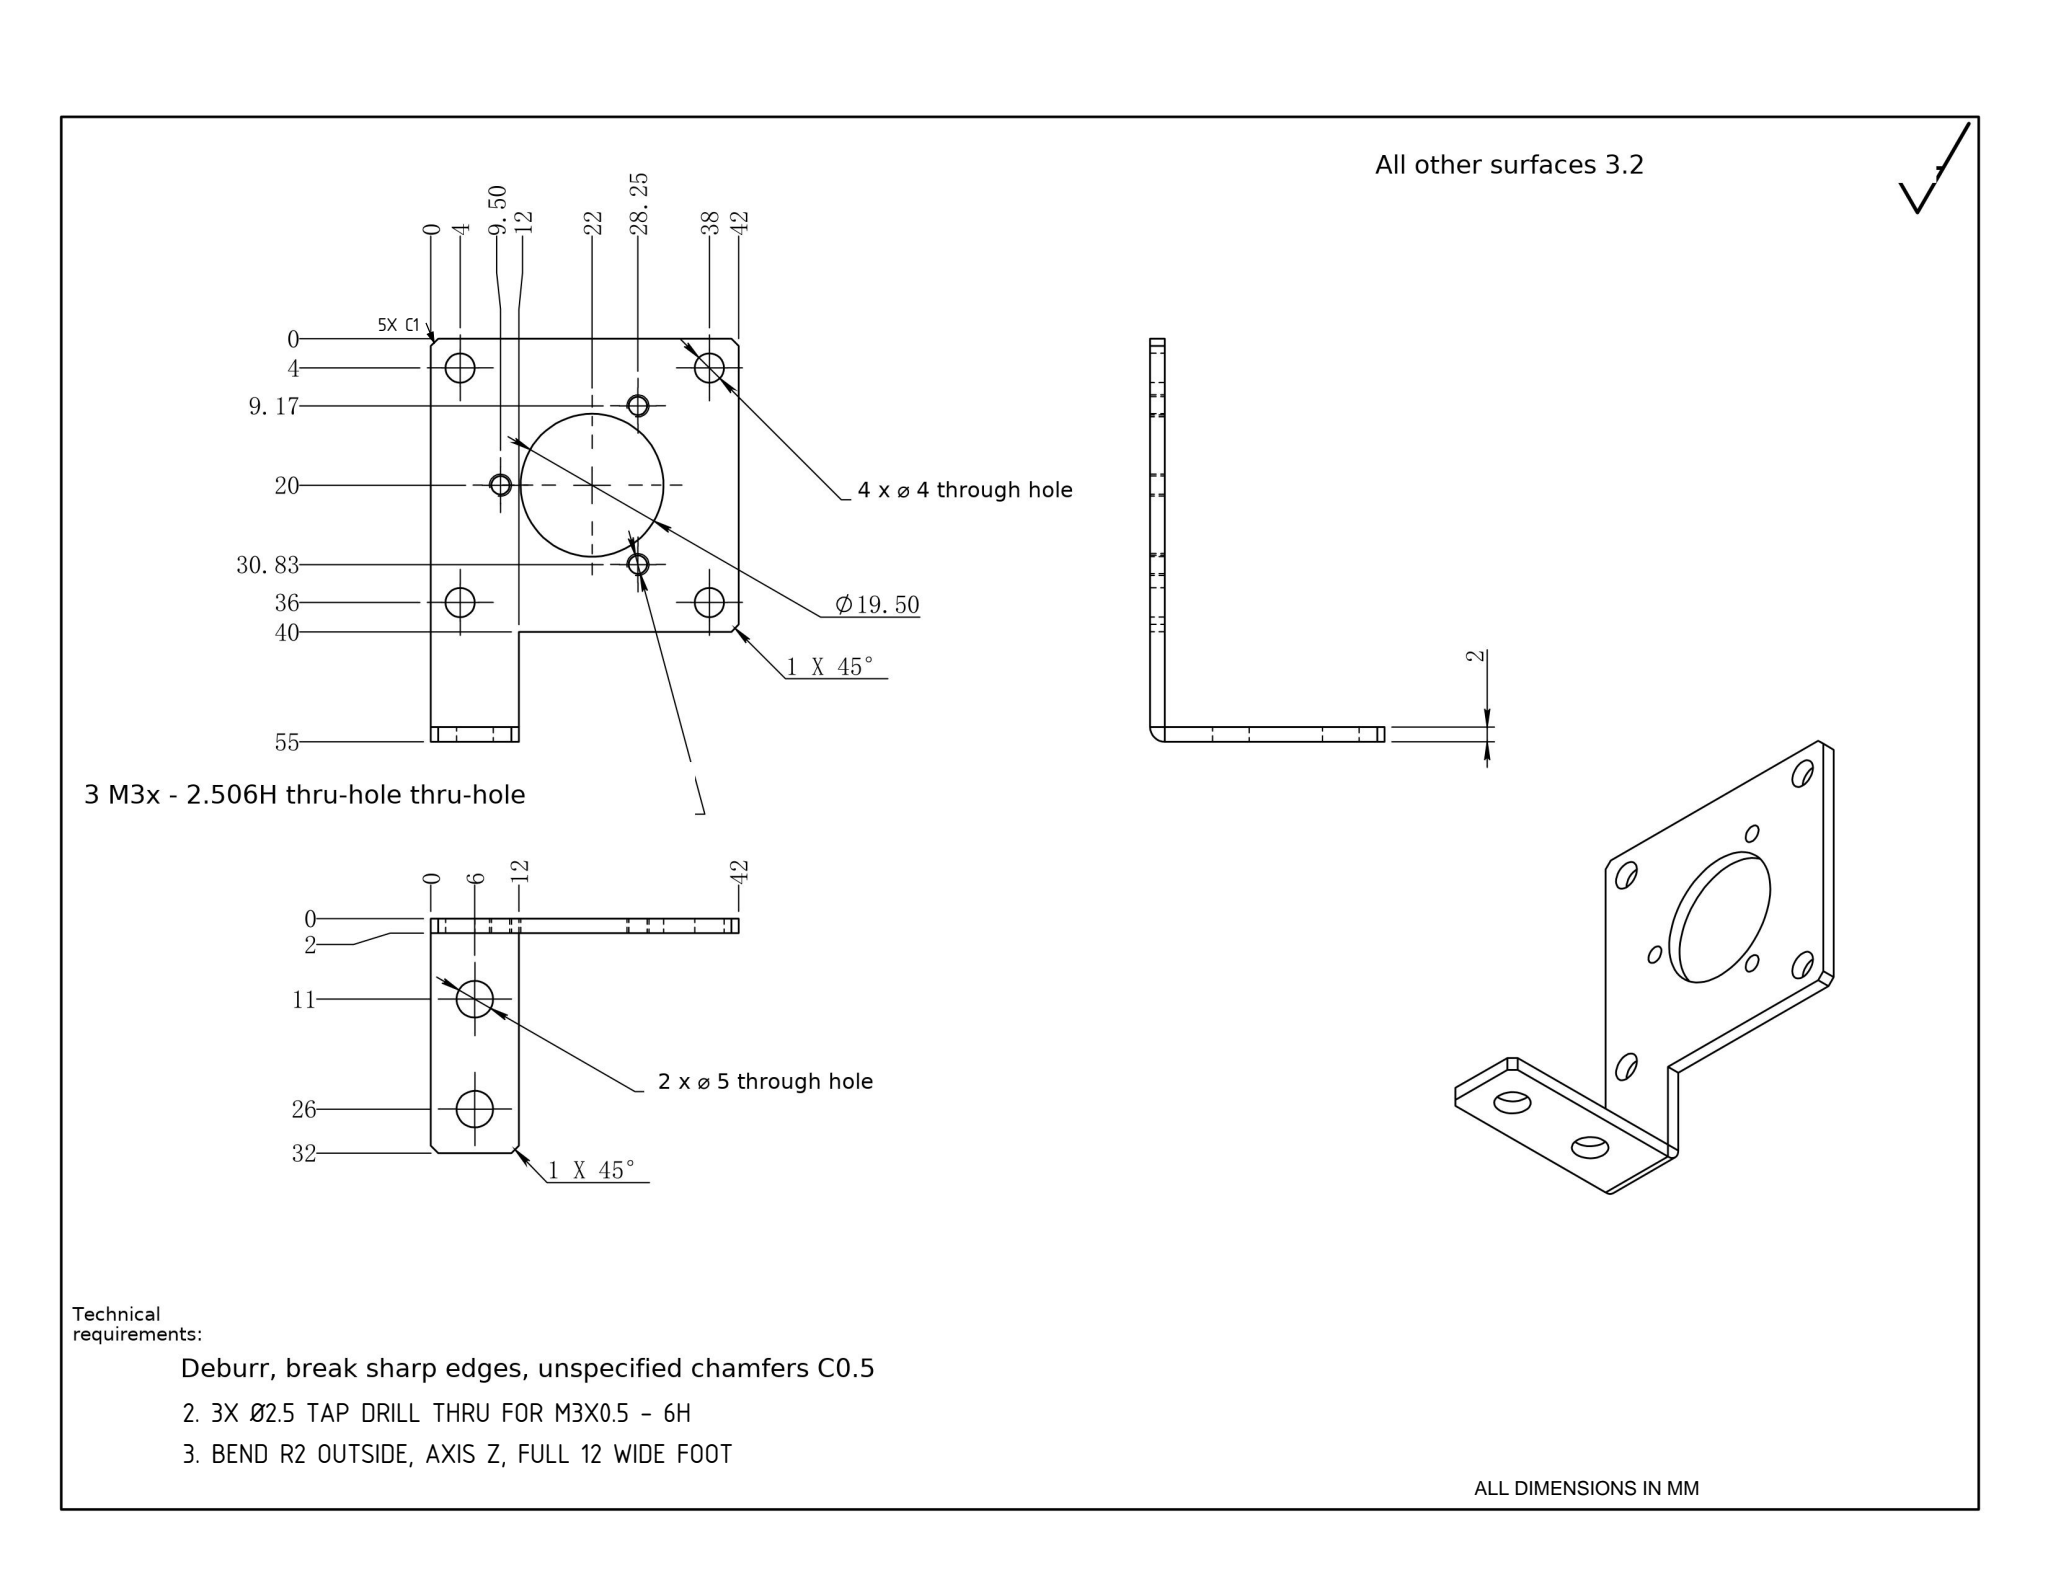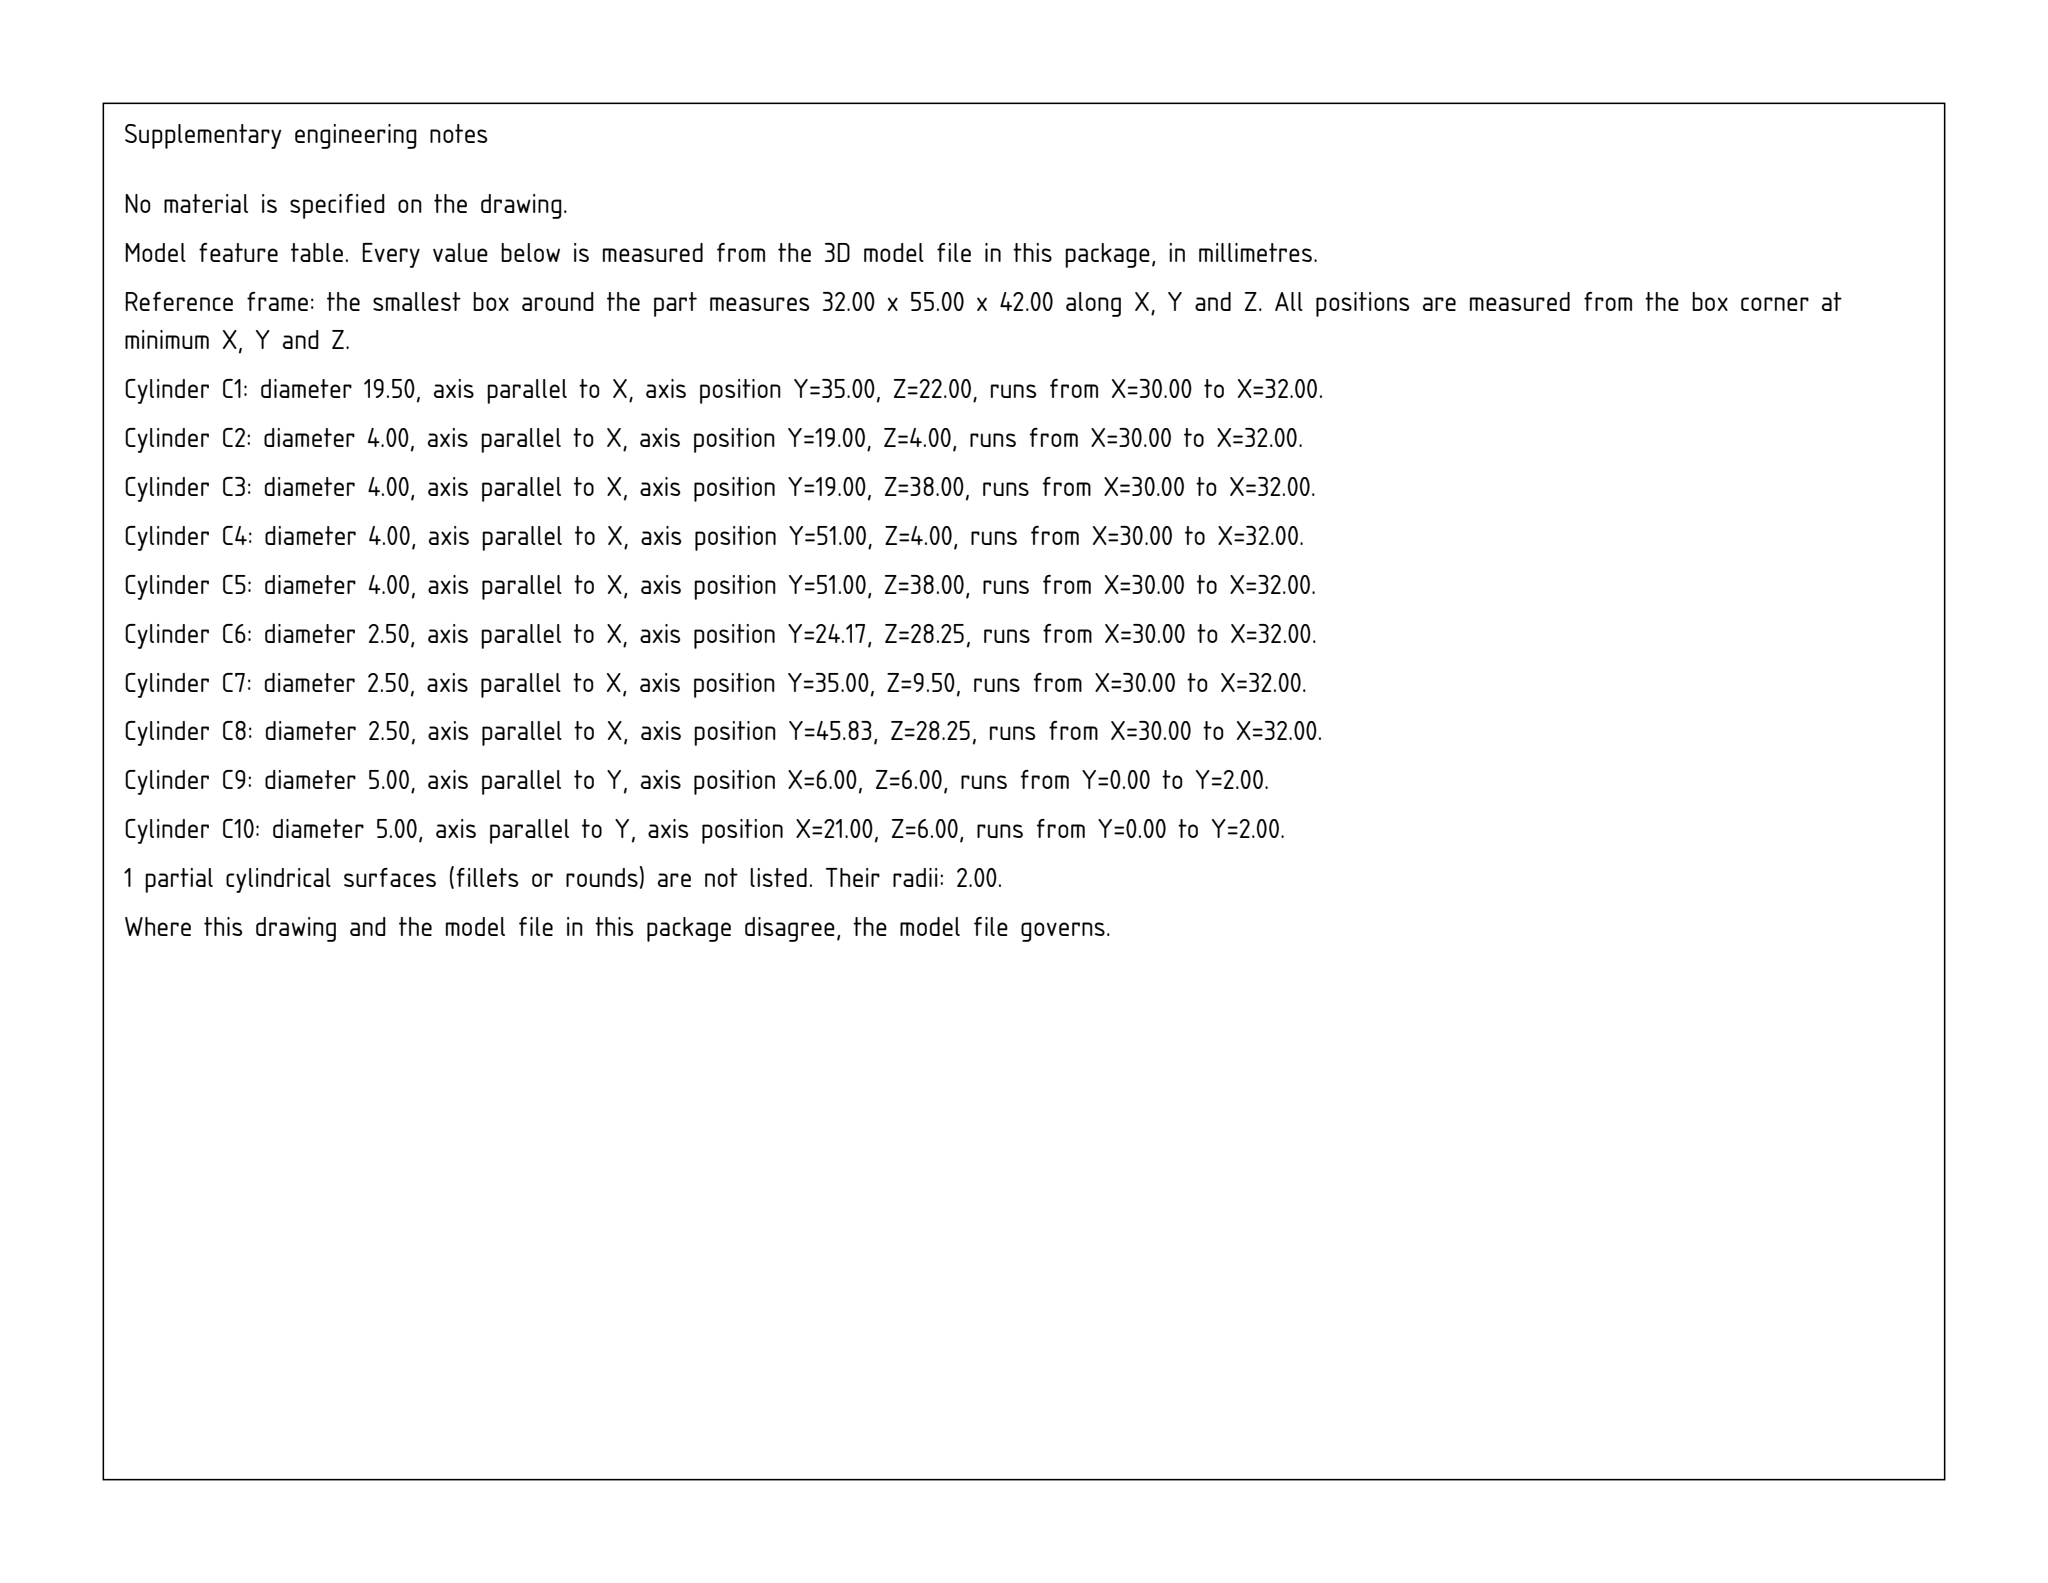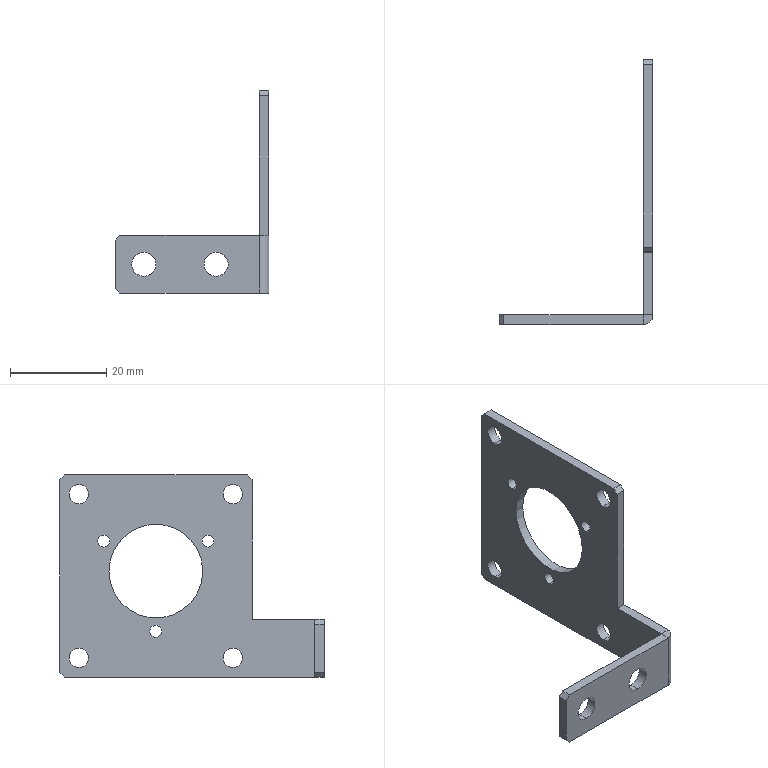Part | SolidWorks | mm | 1 solid | 40 faces | box 32 x 55 x 42 mm | volume 3619 mm3 | cylinder 21 | plane 19 | commonest cylinder face diameters 4 x9 2.5 x6 5 x4 19.5 x2
Drawing notes:
3X Ø2.5 TAP DRILL THRU FOR M3X0.5 - 6H | from the solid: cylinders dia 2.5, axis x, thru 30->32, qty 3 in front plate
BEND R2 OUTSIDE, AXIS Z, FULL 12 WIDE FOOT | from the solid: convex arc dia 4.0 axis z at [30,2], z from 0 to 12 -> R2 outer bend
UNLABELLED 45 CORNERS: 5X C1 (3 ON PLATE, 2 ON FOOT END) | from the solid: 5 inclined planes 45deg, size 1.0 x 1.0: 3 on x=30-32 plate (y15/z41, y54/z0, y54/z41), 2 on foot end x=0 (z0, z11)